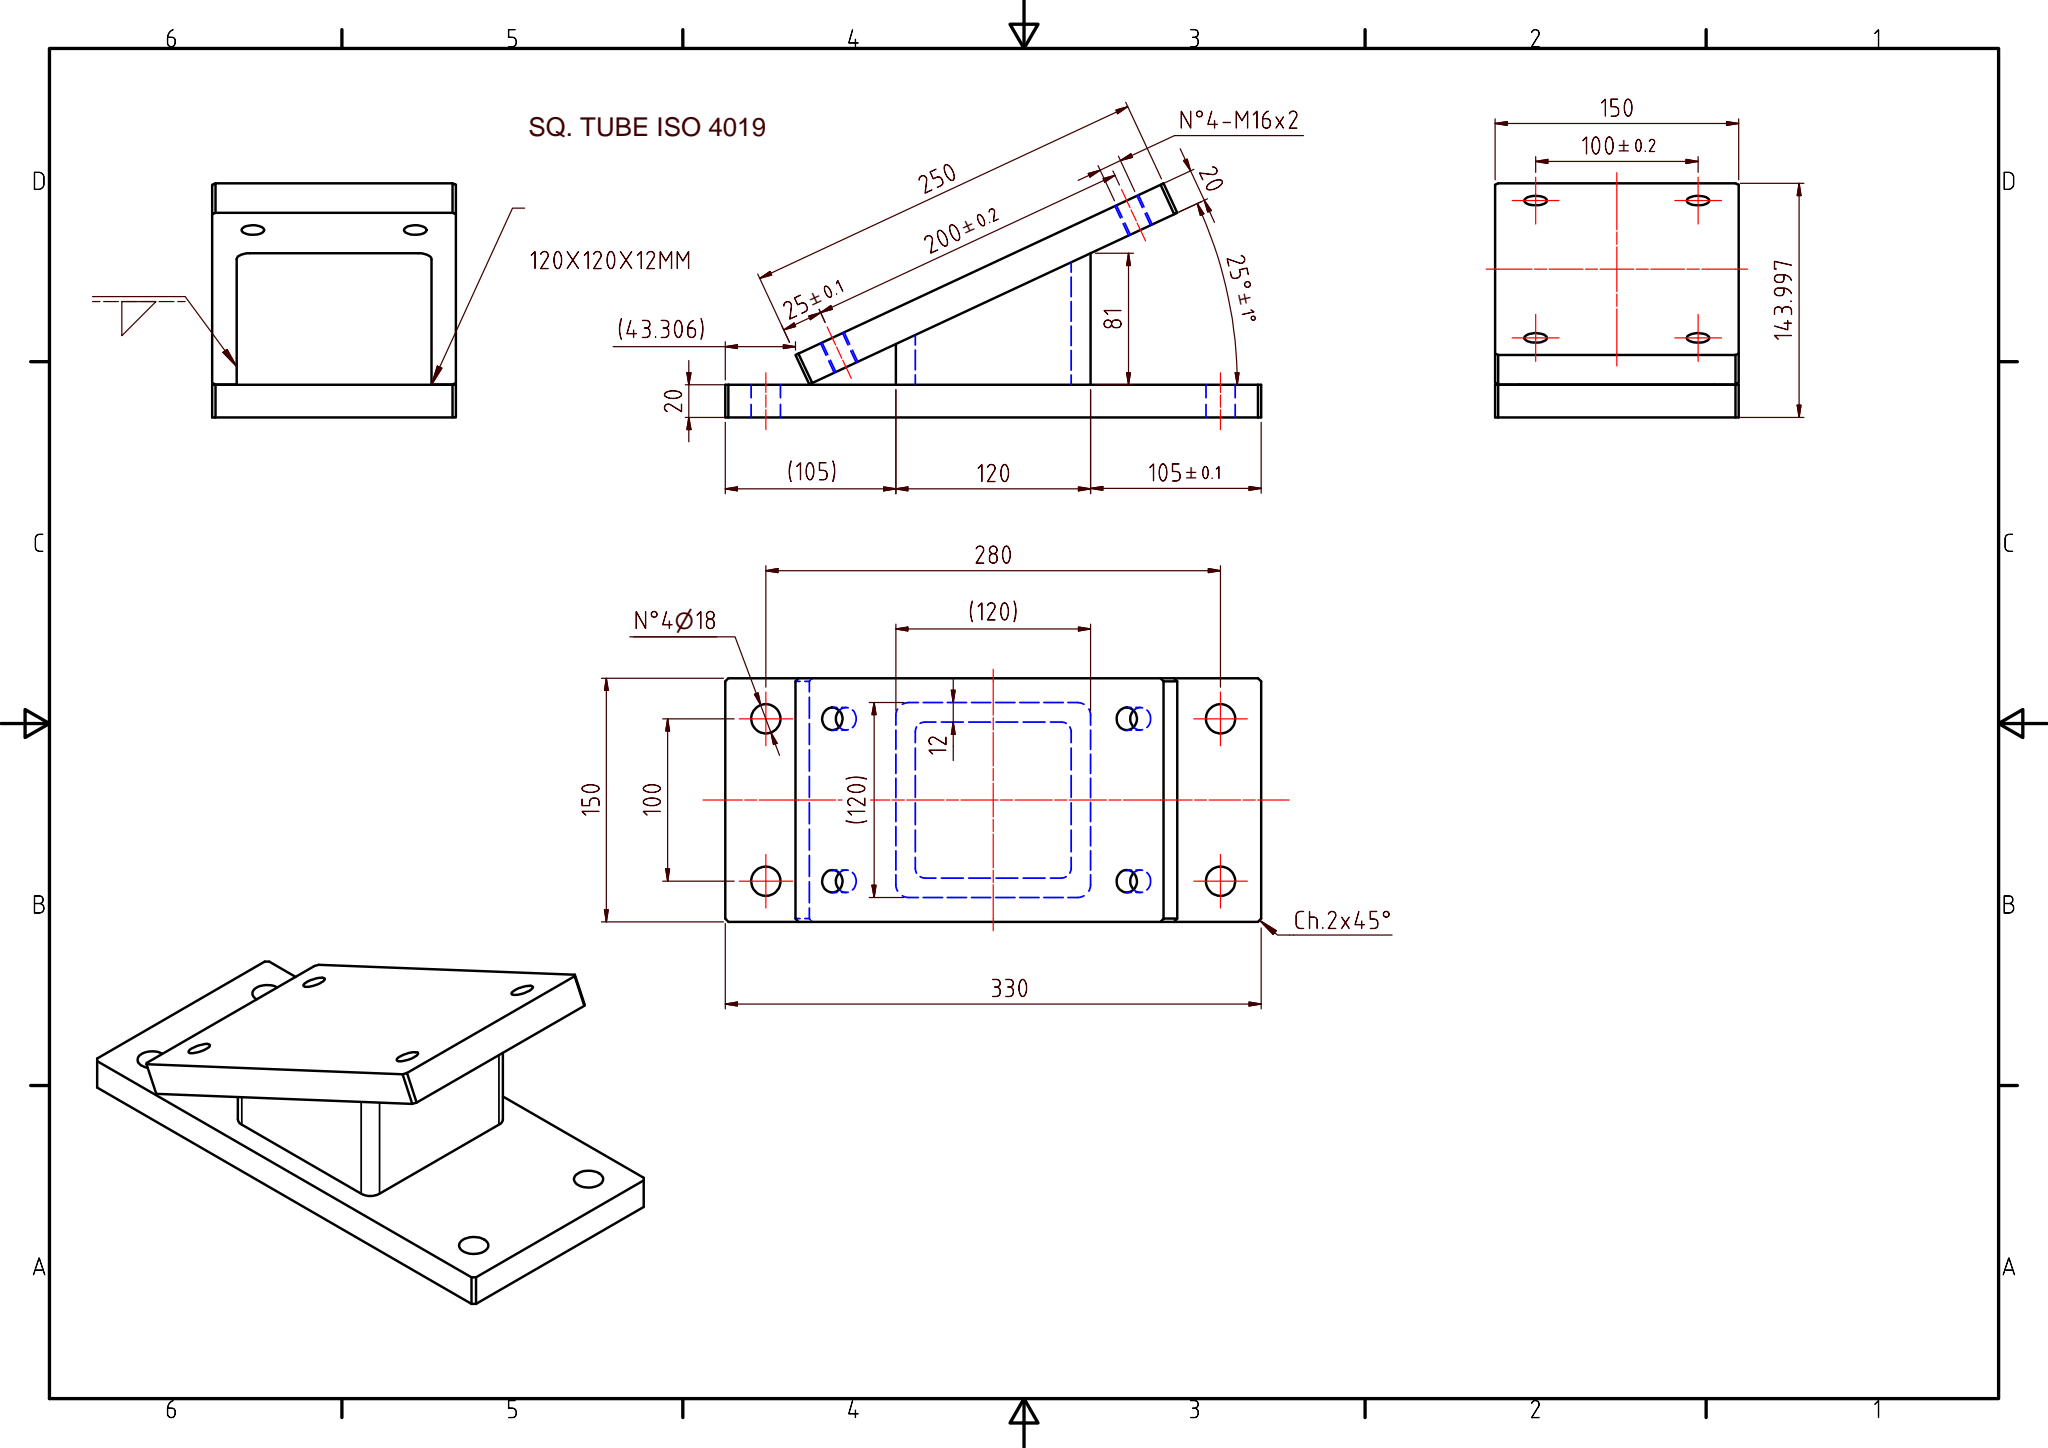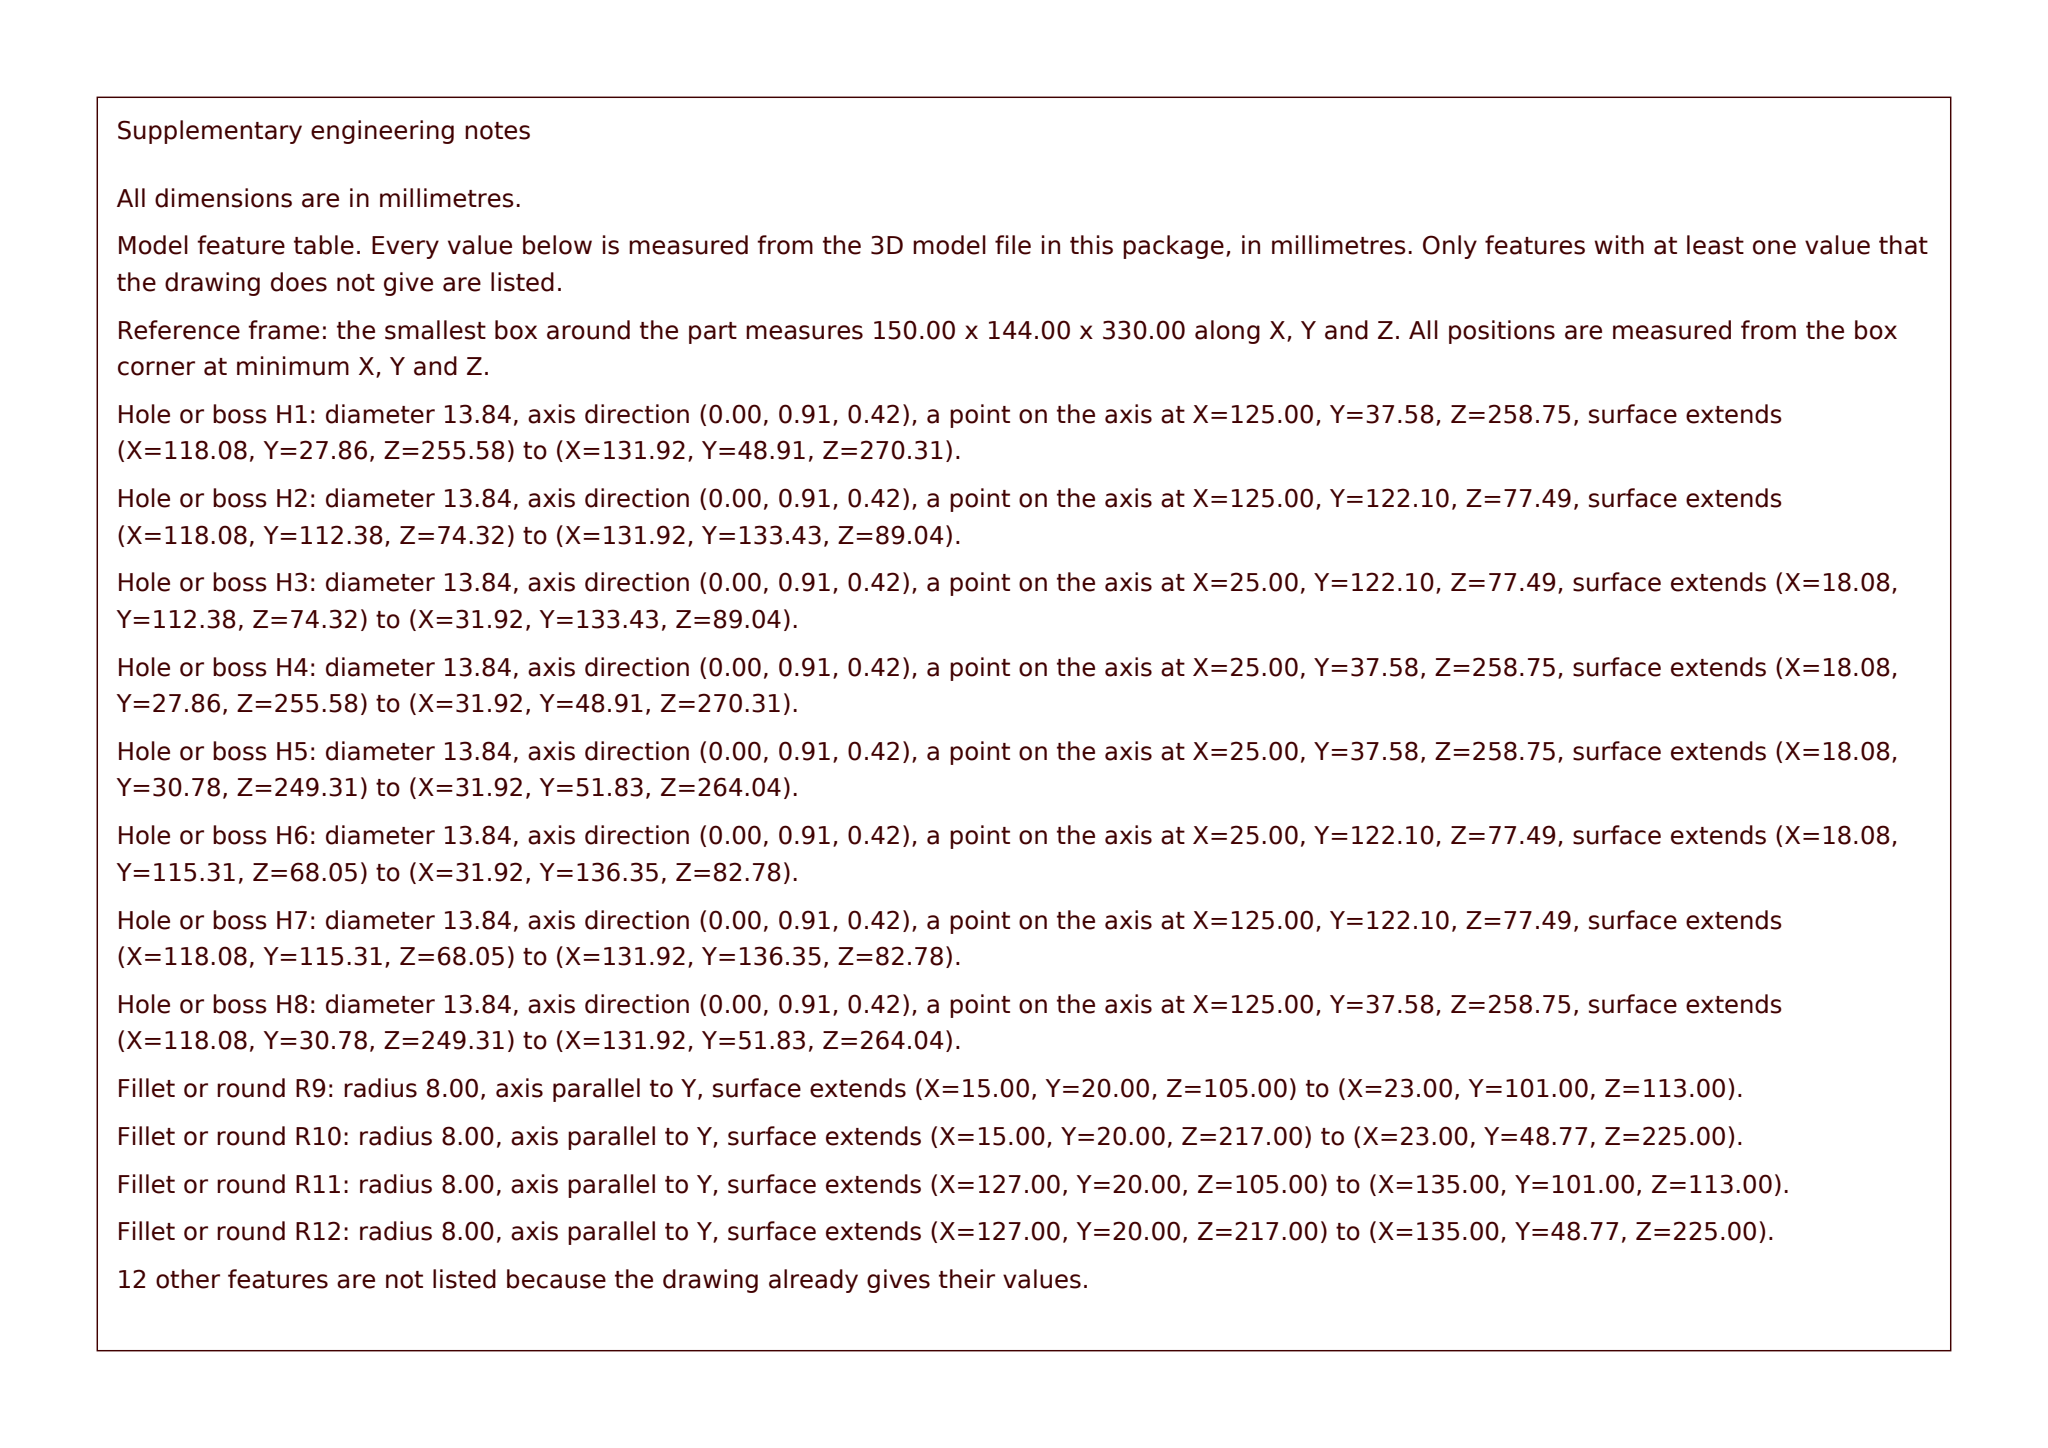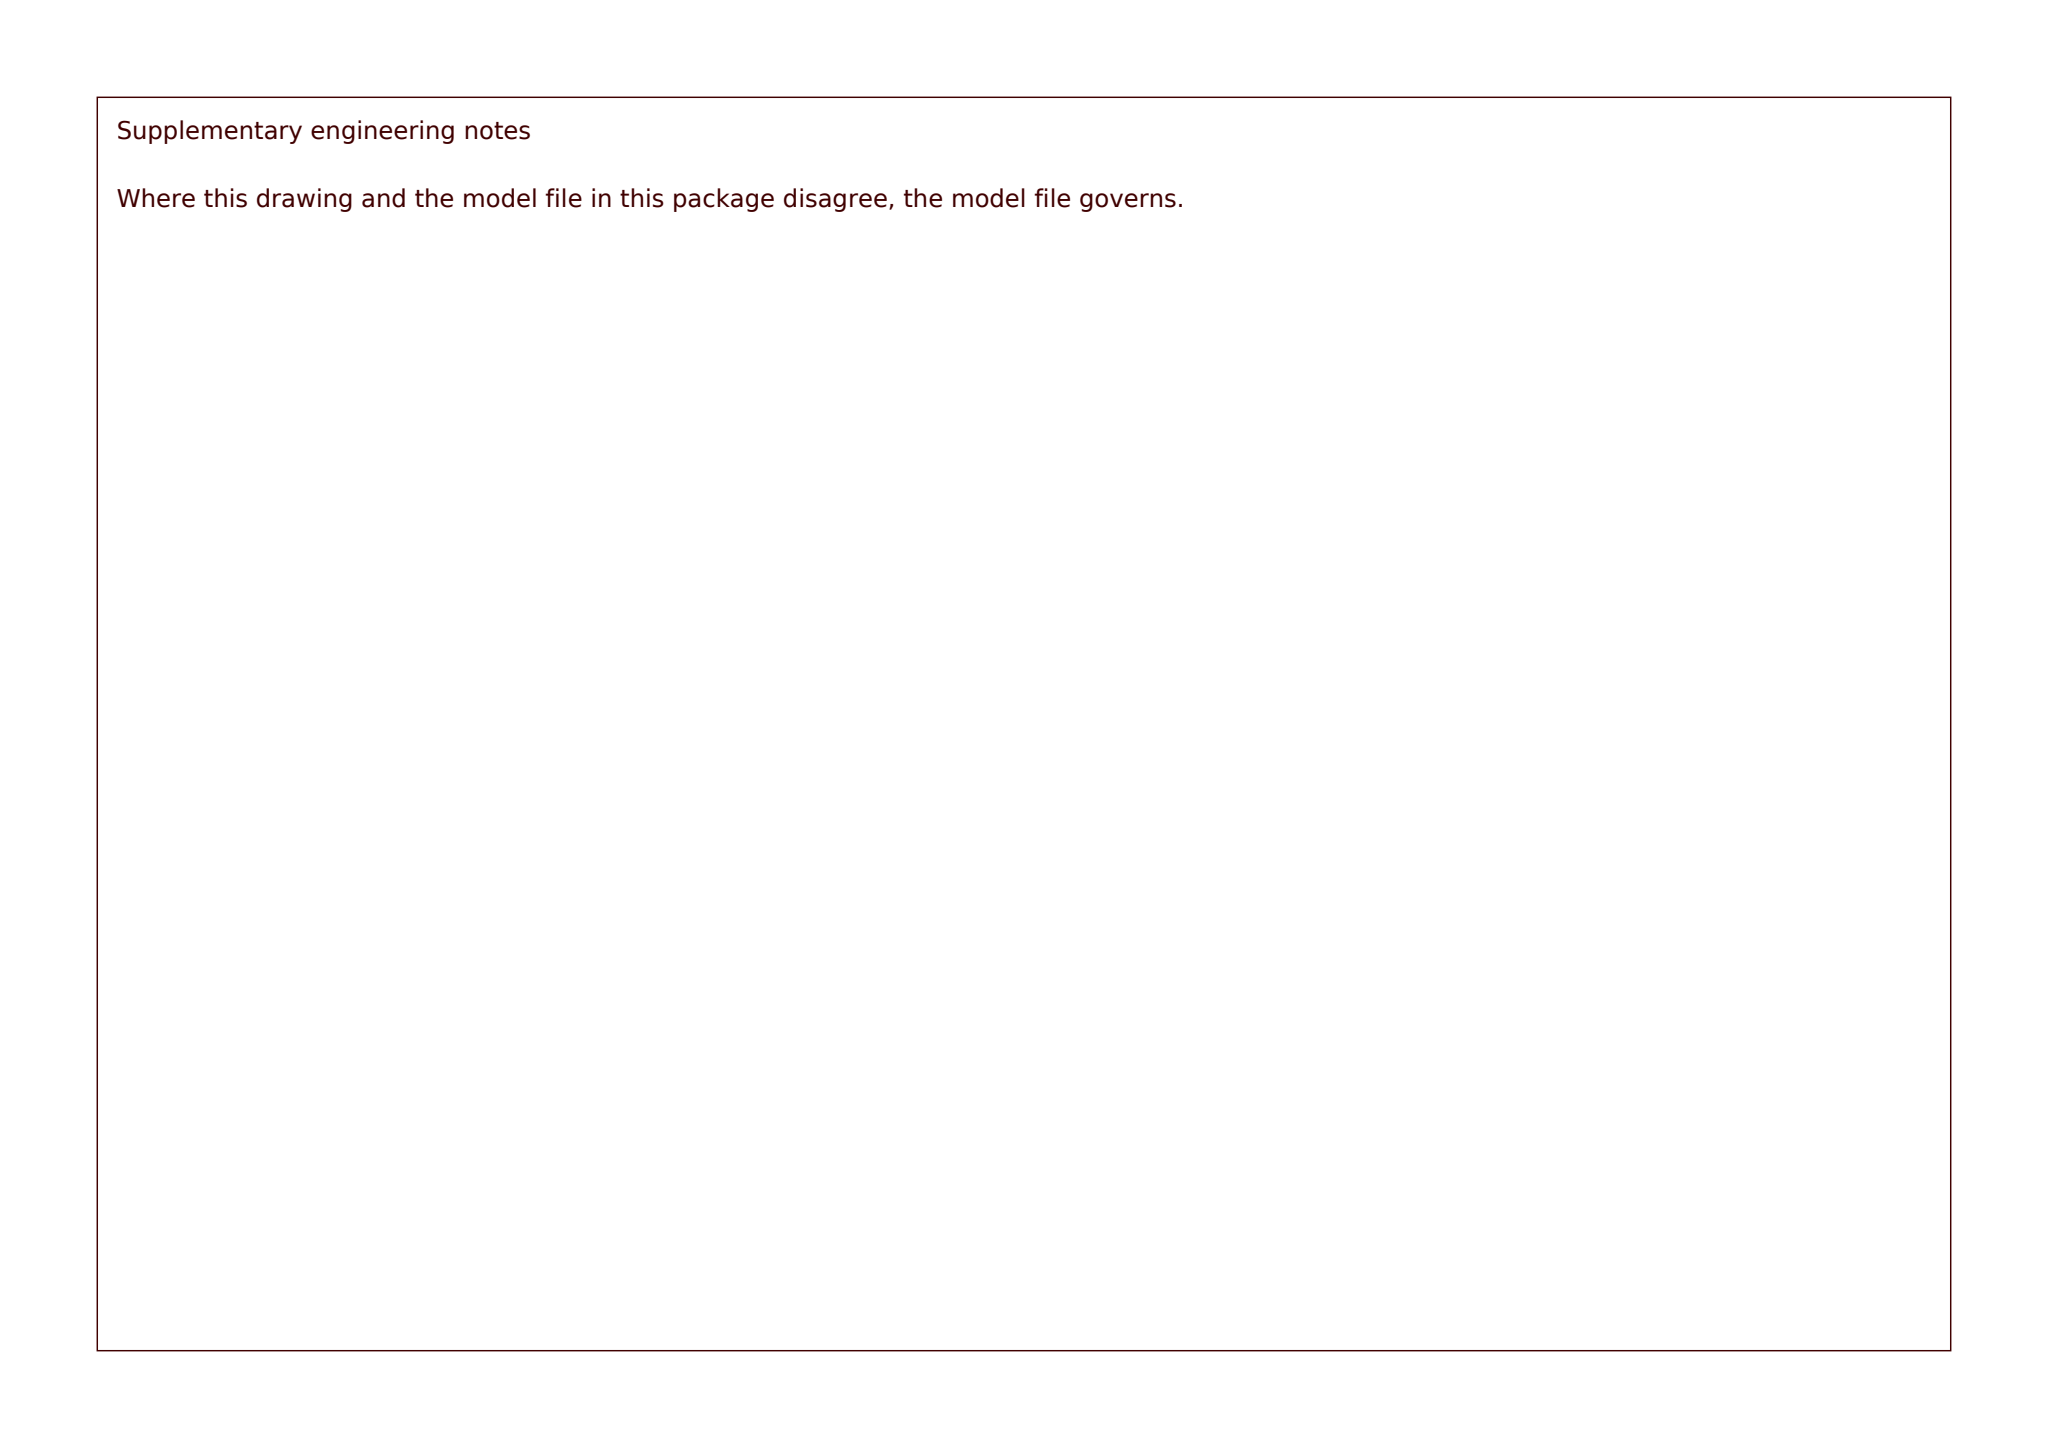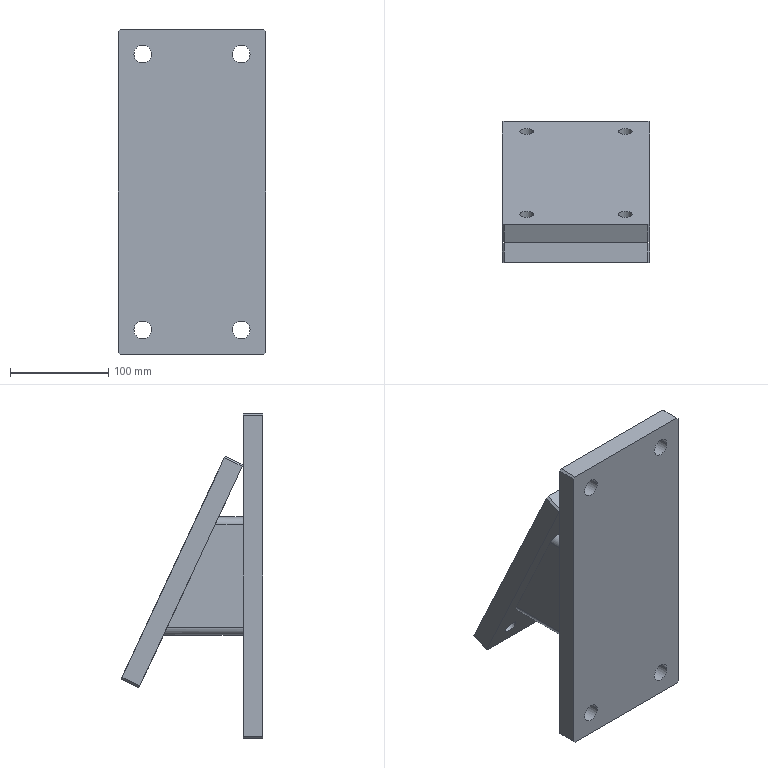Part | SolidWorks | mm | 1 solid | 54 faces | box 150 x 144 x 330 mm | volume 1980885 mm3 | plane 30 | cylinder 24 | commonest cylinder face diameters 18 x8 13.835 x8 16 x4 12 x4